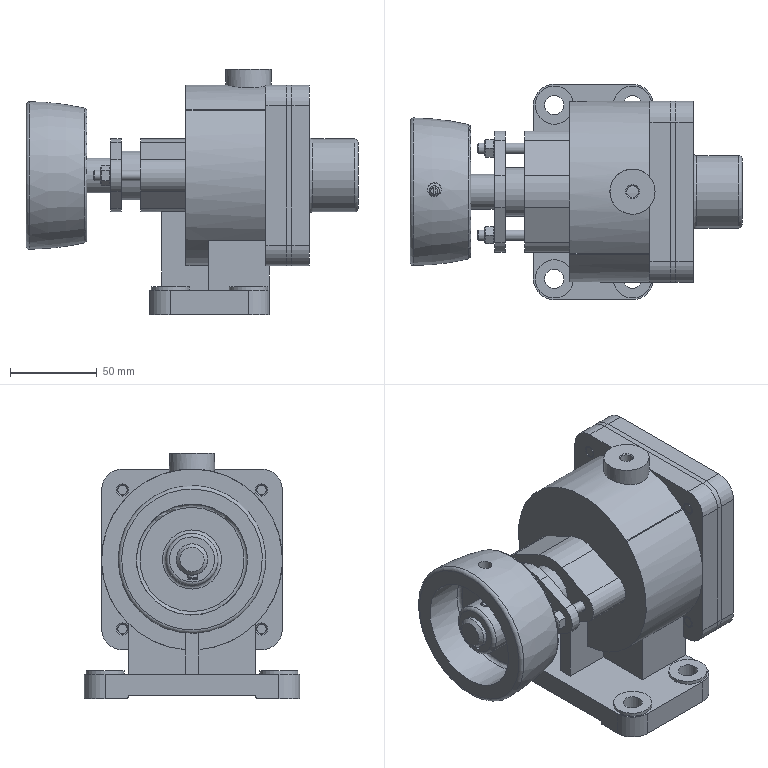Assembly | NX | mm | 21 component files | 21 solids | 355 faces | box 191 x 124 x 141 mm | volume 977637 mm3 | plane 176 | cylinder 115 | cone 53 | torus 9 | spline 2 | commonest cylinder face diameters 6 x20 24 x17 8 x11 20 x9 5 x5 22 x5 42 x5 58 x4
Bill of materials:
unnamed part 1 | 2 |  | Hexagonal prism with a central through-bore; both ends chamfered/crowned so the flats show arched boundaries; raised annular face around the bore at one end. Nut-like shape.
unnamed part 2 | 1 |  | Thin flat square plate with rounded corners, a large central circular opening, and four small holes, one near each corner. Gasket- or flange-plate-like shape.
unnamed part 3 | 1 |  | Short thick-walled cylindrical ring/sleeve with plain ends. It has a radial hole through the outer wall and a small axial hole through the wall at one end face.
unnamed part 4 | 2 |  | Elongated rectangular bar of constant cross-section with one long face slightly convex (curved), the other faces flat.
unnamed part 5 | 2 |  | Solid straight cylindrical rod/pin with small chamfers on both ends.
unnamed part 6 | 1 |  | Square flange plate with rounded corners and four corner through-holes, with a solid cylindrical boss sticking out from the center of one face and a shallow raised pad or step on the opposite face.
unnamed part 7 | 1 |  | Wheel- or pulley-like disc with a slightly crowned outer surface, a recessed face holding a raised central hub, a central bore with one rectangular keyway, and a radial hole in the rim.
unnamed part 8 | 1 |  | Solid cylindrical pin with chamfered or tapered ends on both sides.
unnamed part 9 | 1 |  | Stepped shaft with a large cylindrical collar near one end. The collar has a straight slot cut across its full diameter. The long shaft section has a reduced-diameter end with a small cross hole and a narrow groove/step.
unnamed part 10 | 1 |  | Obround (round-ended rectangular) prism with chamfered edges on top and bottom faces. Resembles a round-ended key.
unnamed part 11 | 4 |  | Headed pin/screw blank: a plain cylindrical shank with a larger cylindrical head that has a chamfered top edge and a straight slot across the head face.
unnamed part 12 | 1 |  | Short headless cylinder with a straight slot across one chamfered end and a conical point at the other end. Resembles a slotted cone-point set screw.
unnamed part 13 | 1 |  | Short thick-walled annular ring with a cylindrical through bore and chamfered outer edges on both end faces.
unnamed part 14 | 1 |  | Housing bracket with a hollow cylindrical body standing on a rectangular base plate. One end has a square flange with rounded corners and four corner holes. There are cylindrical bosses on the top and on one side.
unnamed part 15 | 1 |  | Two-hole flanged sleeve: a flat flange shaped like a rounded diamond or lozenge, with a cylindrical hollow spigot sticking out from one face and a central through bore.
Mates:
1. fix | pump_body 1 component
2. concentric | gasket 1 arc | pump_body 1 edge
3. parallel | gasket 1 face | pump_body 1 face
4. concentric | pump_cover 1 edge | gasket 1 edge
5. parallel | pump_cover 1 face | pump_body 1 face
6. concentric | packing 1 edge | pump_body 1 edge
7. concentric | packing 1 edge | packing_gland 1 edge
8. touch align | packing_gland 1 face | pump_body 1 face
9. parallel | rotor_shaft 1 face | pulley 1 face
10. concentric | pulley 1 edge | rotor_shaft 1 edge
11. concentric | key 1 arc | rotor_shaft 1 edge
12. parallel | key 1 face | rotor_shaft 1 face
13. touch align | screw 1 face | pulley 1 face
14. touch align | screw 1 face | pulley 1 face
15. concentric | screw2 4 | pump_cover 1 edge
16. concentric | screw2 3 | pump_cover 1 edge
17. concentric | screw2 2 edge | pump_cover 1 edge
18. concentric | screw2 1 edge | pump_cover 1 edge
19. touch align | rotor_shaft 1 face | pump_body 1 face
20. concentric | rotor_shaft 1 edge | pump_body 1 edge
21. touch align | eccentric_sleeve 1 face | pump_body 1 face
22. touch align | eccentric_sleeve 1 face | pump_body 1 face
23. center | vane 2 face | vane 2 face | rotor_shaft 1 face | rotor_shaft 1 face
24. touch align | vane 2 face | pump_body 1 face
25. center | vane 1 face | vane 1 face | rotor_shaft 1 face | rotor_shaft 1 face
26. touch align | vane 1 face | pump_body 1 face
27. concentric | pin 1 edge | pump_body 1 edge
28. touch align | stud 2 | pump_body 1 face
29. distance | stud 2 | packing_gland 1 face
30. touch align | stud 1 face | packing_gland 1 face
31. distance | stud 1 face | packing_gland 1 face
32. concentric | nut 2 | packing_gland 1 edge
33. concentric | nut 1 edge | packing_gland 1 edge